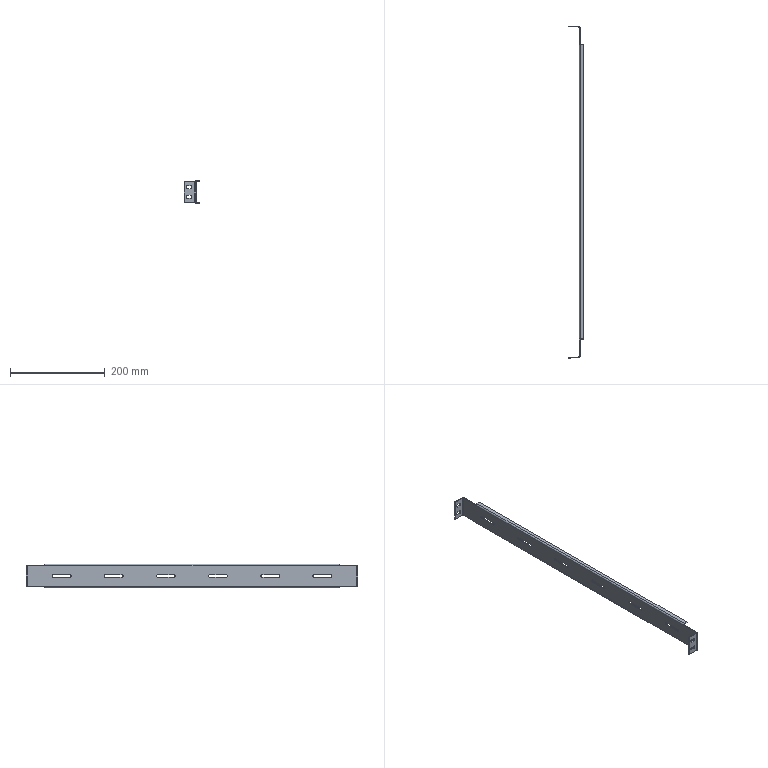Component | SolidWorks | RailMountingBeam-11 | 1 solid | 88 faces | volume 87725 mm3 | plane 50 | cylinder 38 | commonest cylinder face diameters 5 x18 7 x12 6 x4 2 x4